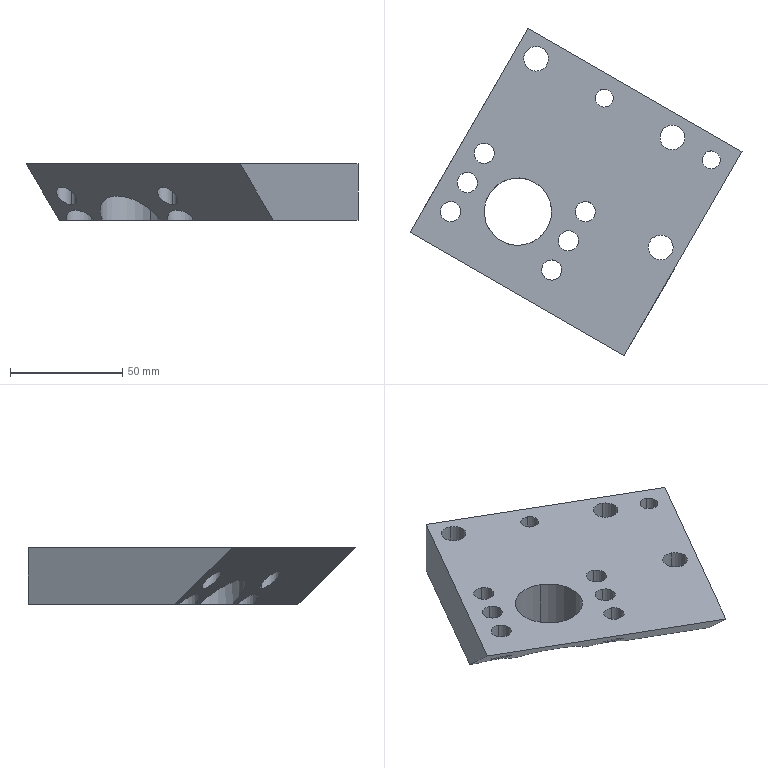Component | SolidWorks | KLHFH008LimitPlate-SymmetricPart-1 | 1 solid | 45 faces | box 147.76 x 145.93 x 25 mm | volume 205141 mm3 | cylinder 34 | plane 11 | commonest cylinder face diameters 9 x12 18 x6 11 x6 8 x4 15 x4 30 x2 | material Plain Carbon Steel
build123d program:
from build123d import *

# Parameters (mm, degrees)
SKETCH1_W                                         = 110
SKETCH1_H                                         = 110
BOSS_EXTRUDE1_DEPTH                               = 12.5
HOLE_SIZE_ACCORDING_TO_TYPE_OF_HEXAGO_D           = 11
HOLE_SIZE_ACCORDING_TO_TYPE_OF_HEXAGO_CBORE_D     = 18
HOLE_SIZE_ACCORDING_TO_TYPE_OF_HEXAGO_CBORE_DEPTH = 11
F_9_0_9_DIAMETER_HOLE1_D                          = 9
HOLE1_D                                           = 9
HOLE1_CBORE_D                                     = 15
HOLE1_CBORE_DEPTH                                 = 15
SIZE_MM_DOWEL_PIN_HOLE2_D                         = 8
SKETCH10_R                                        = 15
CUT_EXTRUDE1_DEPTH                                = 82.701
CUT_EXTRUDE2_DEPTH                                = 124.617


with BuildPart() as part:
    # Sketch1 → Boss-Extrude1 (new, symmetric)
    with BuildSketch(Plane.XY):
        Rectangle(SKETCH1_W, SKETCH1_H)
    extrude(amount=BOSS_EXTRUDE1_DEPTH, both=True)

    # Hole Size _ according to_ Type of Hexago (through all)
    with Locations(Plane(origin=(0, 0, -12.5), x_dir=(1, 0, 0), z_dir=(0, 0, -1))):
        with Locations((44.992, 25), (45, -45), (0, 45)):
            CounterBoreHole(HOLE_SIZE_ACCORDING_TO_TYPE_OF_HEXAGO_D / 2, HOLE_SIZE_ACCORDING_TO_TYPE_OF_HEXAGO_CBORE_D / 2, HOLE_SIZE_ACCORDING_TO_TYPE_OF_HEXAGO_CBORE_DEPTH)

    # 9.0 _9_ Diameter Hole1 (through all)
    with Locations(Plane.XY.offset(12.5)):
        with Locations((-33, 43.981), (-3, 43.981), (-3, -7.981), (-33, -7.981)):
            Hole(F_9_0_9_DIAMETER_HOLE1_D / 2)

    # Hole1 (through all)
    with Locations(Plane(origin=(0, 0, -12.5), x_dir=(1, 0, 0), z_dir=(0, 0, -1))):
        with Locations((-18, -43.981), (-18, 7.981)):
            CounterBoreHole(HOLE1_D / 2, HOLE1_CBORE_D / 2, HOLE1_CBORE_DEPTH)

    # Size mm Dowel Pin Hole2 (through all)
    with Locations(Plane.XY.offset(12.5)):
        with Locations((44.996, 10), (44.99, -45)):
            Hole(SIZE_MM_DOWEL_PIN_HOLE2_D / 2)

    # Sketch10 → Cut-Extrude1 (cut, through all)
    with BuildSketch(Plane.XY.offset(12.5)):
        with Locations((-18, 18)):
            Circle(SKETCH10_R)
    extrude(amount=-CUT_EXTRUDE1_DEPTH, mode=Mode.SUBTRACT)

    # Sketch11 → Cut-Extrude2 (cut, through all)
    with BuildSketch(Plane.XZ.offset(55)):
        Polygon((-55, 12.5), (-50, 12.5), (-20.206, -12.5), (-55, -12.5), align=None)
    extrude(amount=-CUT_EXTRUDE2_DEPTH, mode=Mode.SUBTRACT)


solid = part.part

# Placed as in the assembly
solid = solid.moved(Location((115.588, 164.205, -456.5), (0, 0, 60)))